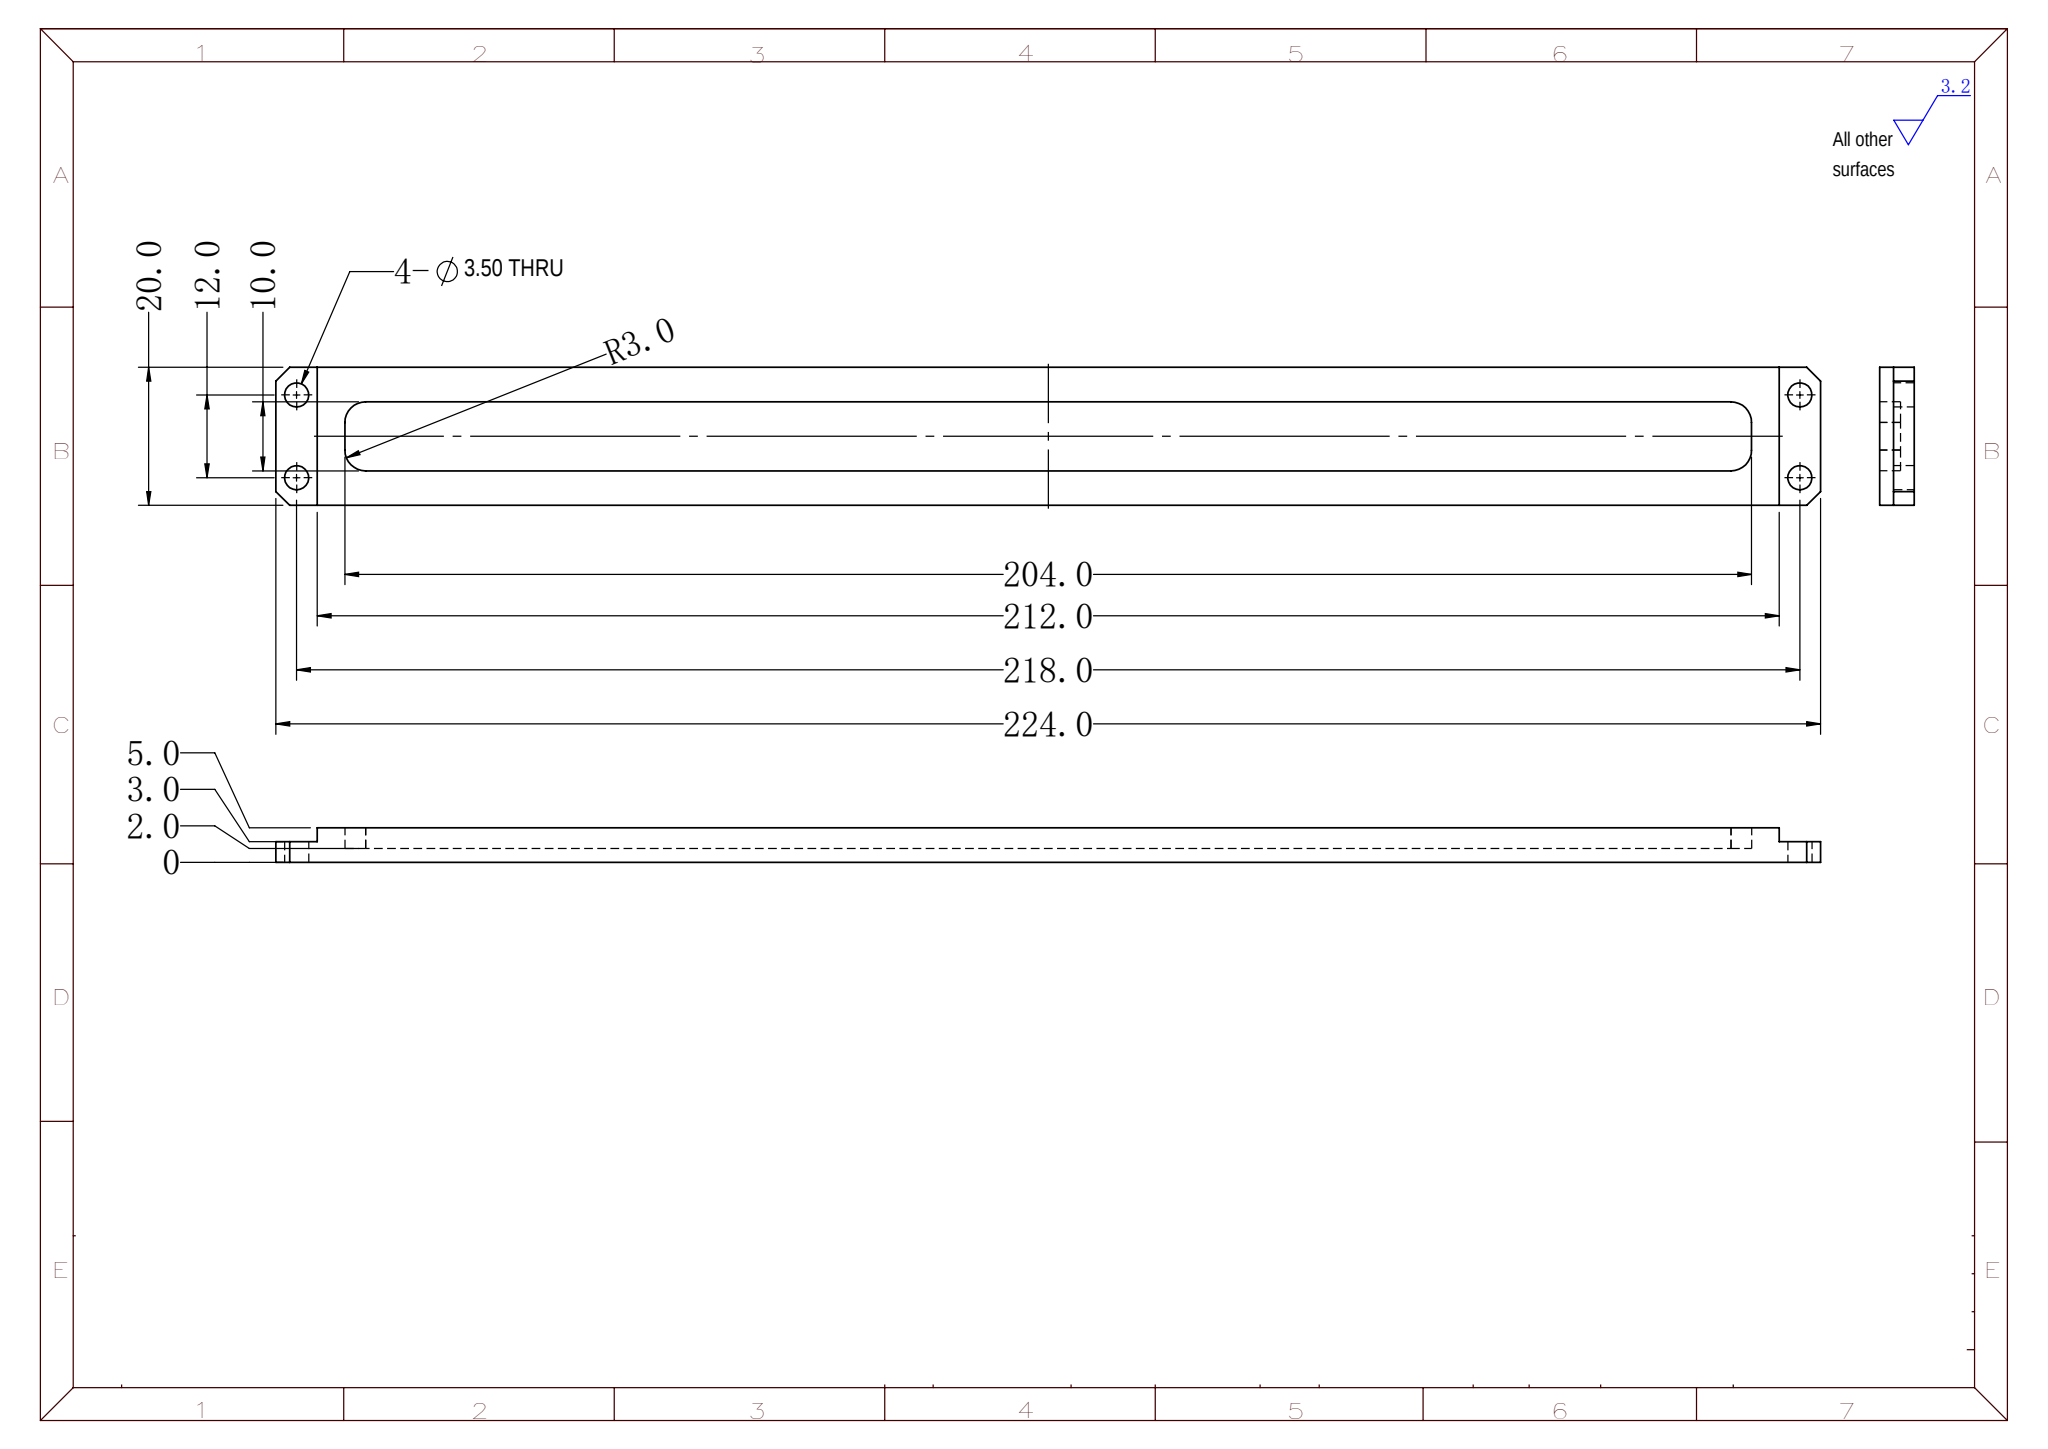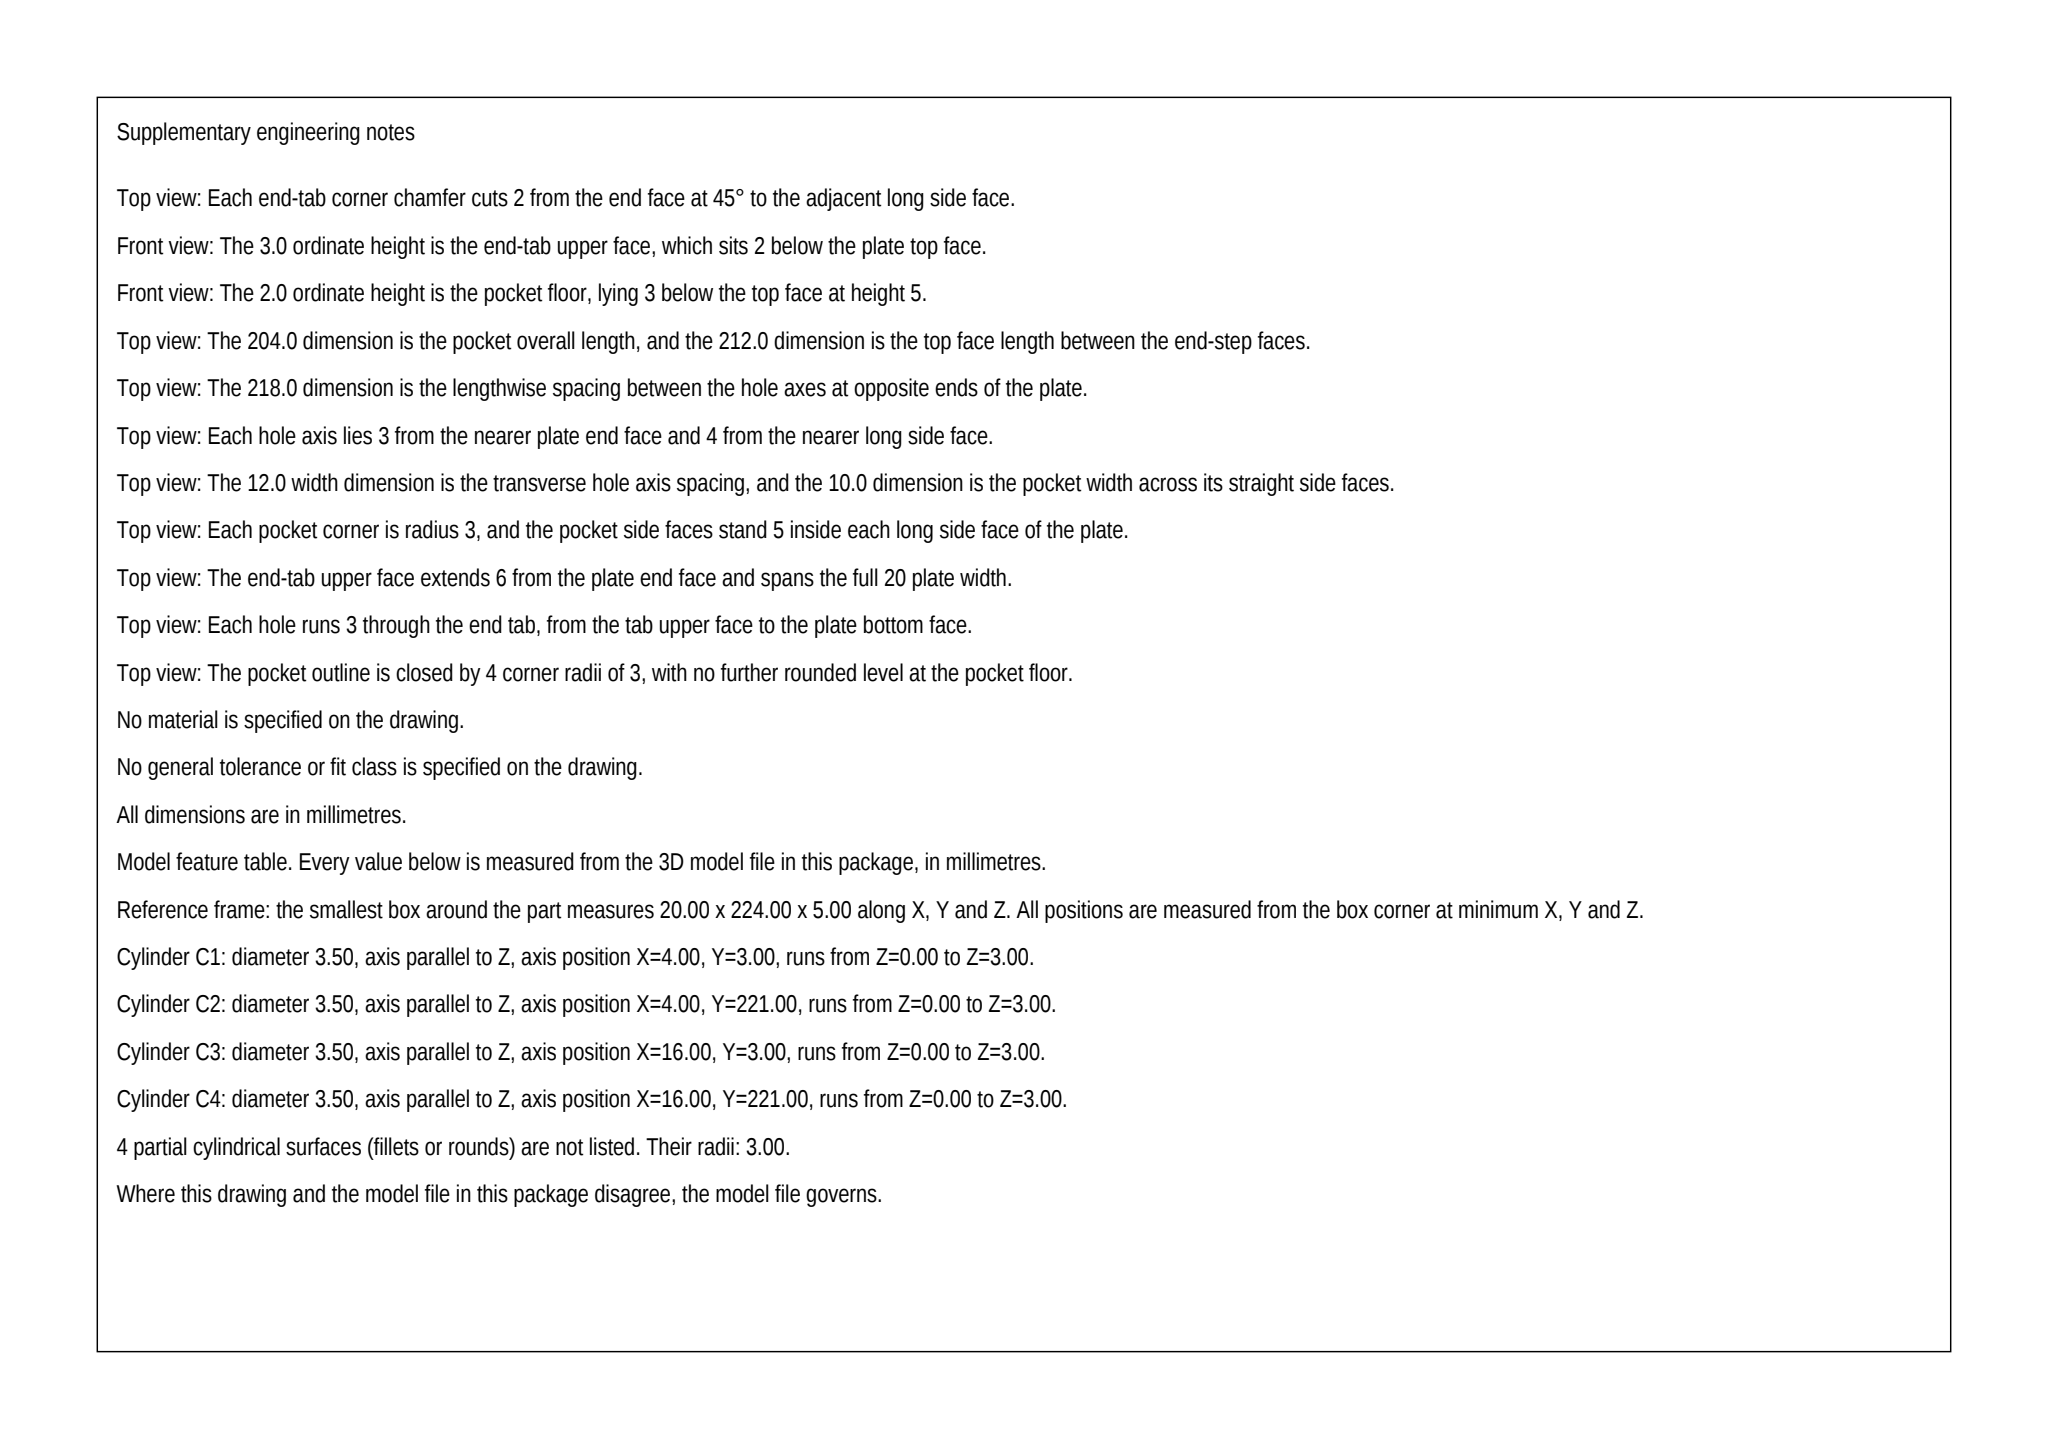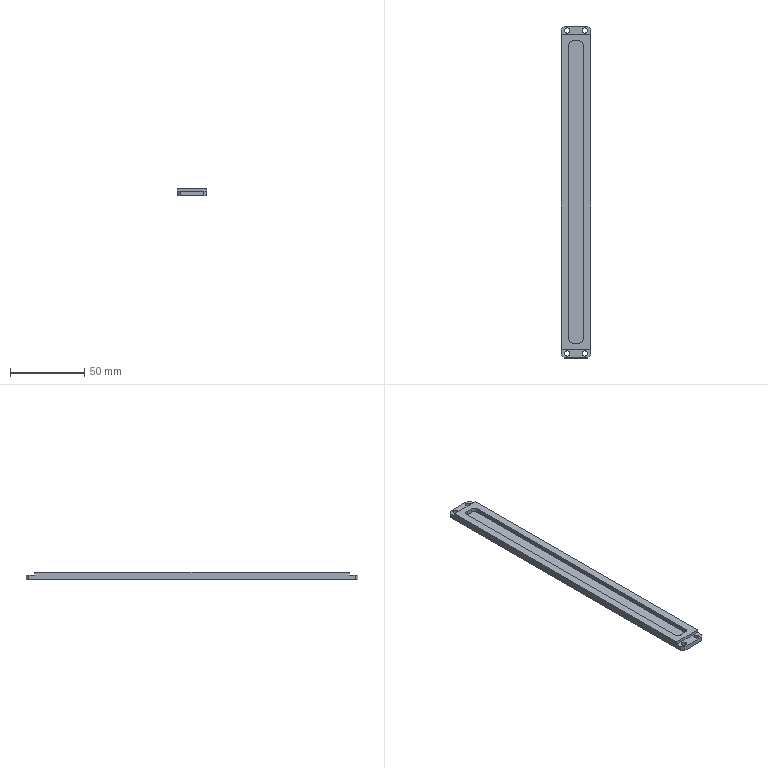Part | SolidWorks | mm | 1 solid | 31 faces | box 20 x 224 x 5 mm | volume 15684 mm3 | plane 19 | cylinder 12 | commonest cylinder face diameters 3.5 x8 6 x4
Drawing notes:
END PAD CORNERS: CHAM 5 X 4 (4 ACROSS LENGTH), 4 PLCS | from the solid: x-planes 0/5/15/20 & y-planes 0/6/10/214/218/224: pad 20 wide tapers to 10 wide body over y 6->10, i.e. 5 in X by 4 in Y at each of 4 corners
build123d program:
from build123d import *

# Parameters (mm, degrees)
SKETCH1_W           = 20
SKETCH1_H           = 224
BOSS_EXTRUDE1_DEPTH = 5
SKETCH2_W           = 37.667
SKETCH2_H           = 6
CUT_EXTRUDE1_DEPTH  = 2
SKETCH3_R           = 1.75
CUT_EXTRUDE2_DEPTH  = 10
CHAMFER1_SIZE       = 2
CUT_EXTRUDE3_DEPTH  = 3


with BuildPart() as part:
    # Sketch1 → Boss-Extrude1 (new body)
    with BuildSketch(Plane.XY):
        Rectangle(SKETCH1_W, SKETCH1_H)
    extrude(amount=BOSS_EXTRUDE1_DEPTH)

    # Sketch2 → Cut-Extrude1 (cut)
    with BuildSketch(Plane.XY.offset(5)):
        with Locations((-0.6248, 109)):
            Rectangle(SKETCH2_W, SKETCH2_H)
    cut_extrude1 = extrude(amount=-CUT_EXTRUDE1_DEPTH, mode=Mode.SUBTRACT)

    # Sketch3 → Cut-Extrude2 (cut)
    with BuildSketch(Plane(origin=(0, 0, 0), x_dir=(-1, 0, 0), z_dir=(0, 0, -1))):
        with Locations((-6, -109)):
            Circle(SKETCH3_R)
        with Locations((6, -109)):
            Circle(SKETCH3_R)
    cut_extrude2 = extrude(amount=-CUT_EXTRUDE2_DEPTH, mode=Mode.SUBTRACT)

    # Mirror1: Cut-Extrude2 across plane
    add(cut_extrude2.mirror(Plane.ZX), mode=Mode.SUBTRACT)

    # Mirror2: Cut-Extrude1 across plane
    add(cut_extrude1.mirror(Plane.ZX), mode=Mode.SUBTRACT)

    # Chamfer1
    chamfer1_edges = [part.edges().sort_by_distance(p)[0] for p in [
        (-10, 112, 1.5),
        (10, 112, 1.5),
        (10, -112, 1.5),
        (-10, -112, 1.5),
    ]]
    chamfer(chamfer1_edges, length=CHAMFER1_SIZE)

    # Sketch4 → Cut-Extrude3 (cut)
    with BuildSketch(Plane.XY.offset(5)):
        with BuildLine():
            Line((-2, -102), (2, -102))
            ThreePointArc((2, -102), (4.121, -101.121), (5, -99))
            Line((5, -99), (5, 99))
            ThreePointArc((5, 99), (4.121, 101.121), (2, 102))
            Line((2, 102), (-2, 102))
            ThreePointArc((-2, 102), (-4.121, 101.121), (-5, 99))
            Line((-5, 99), (-5, -99))
            ThreePointArc((-5, -99), (-4.121, -101.121), (-2, -102))
        make_face()
    extrude(amount=-CUT_EXTRUDE3_DEPTH, mode=Mode.SUBTRACT)


solid = part.part